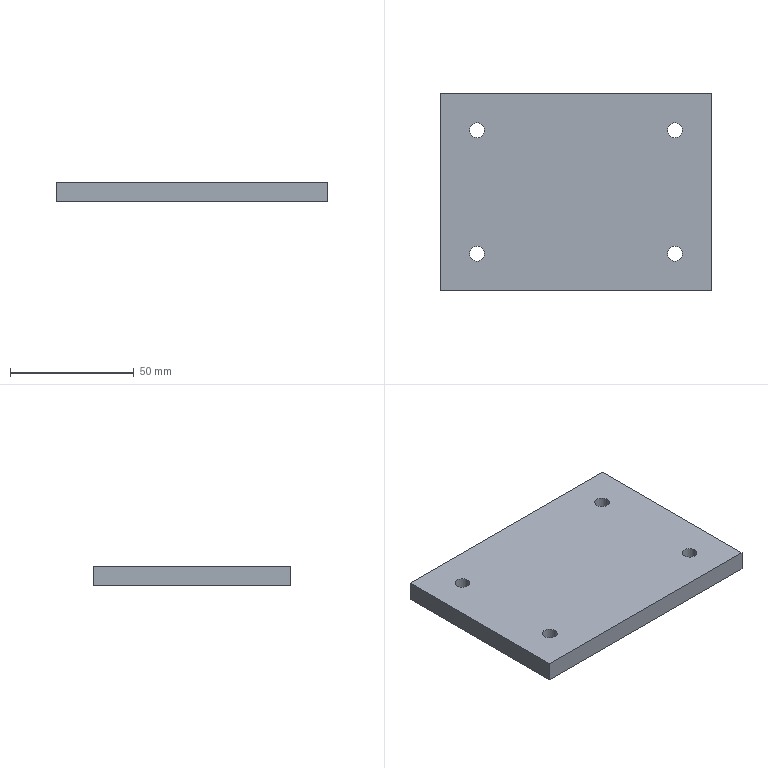Component | NX | 5 | 1 solid | 10 faces | box 110 x 80 x 8 mm | volume 69495 mm3 | plane 6 | cylinder 4 | commonest cylinder face diameters 6 x4
STEP:
#1=CARTESIAN_POINT('',(0.,0.,0.));
#2=DIRECTION('',(0.,0.,1.));
#3=DIRECTION('',(1.,0.,0.));
#4=AXIS2_PLACEMENT_3D('',#1,#2,#3);
#5=CARTESIAN_POINT('',(-55.,40.,0.));
#6=VERTEX_POINT('',#5);
#7=CARTESIAN_POINT('',(-55.,-40.,0.));
#8=VERTEX_POINT('',#7);
#9=CARTESIAN_POINT('',(-55.,40.,0.));
#10=DIRECTION('',(-0.,-1.,0.));
#11=VECTOR('',#10,1.);
#12=LINE('',#9,#11);
#13=CARTESIAN_POINT('',(-55.,40.,-8.));
#14=DIRECTION('',(-1.,0.,0.));
#15=DIRECTION('',(-0.,-1.,0.));
#16=AXIS2_PLACEMENT_3D('',#13,#14,#15);
#17=PLANE('',#16);
#18=CARTESIAN_POINT('',(0.,8.));
#19=DIRECTION('',(1.,0.));
#20=VECTOR('',#19,1.);
#21=LINE('',#18,#20);
#22=(GEOMETRIC_REPRESENTATION_CONTEXT(2)PARAMETRIC_REPRESENTATION_CONTEXT()REPRESENTATION_CONTEXT('',''));
#23=DEFINITIONAL_REPRESENTATION('',(#21),#22);
#24=PCURVE('',#17,#23);
#25=CARTESIAN_POINT('',(0.,0.,0.));
#26=DIRECTION('',(0.,0.,1.));
#27=DIRECTION('',(1.,0.,0.));
#28=AXIS2_PLACEMENT_3D('',#25,#26,#27);
#29=PLANE('',#28);
#30=CARTESIAN_POINT('',(-55.,40.));
#31=DIRECTION('',(-0.,-1.));
#32=VECTOR('',#31,1.);
#33=LINE('',#30,#32);
#34=(GEOMETRIC_REPRESENTATION_CONTEXT(2)PARAMETRIC_REPRESENTATION_CONTEXT()REPRESENTATION_CONTEXT('',''));
#35=DEFINITIONAL_REPRESENTATION('',(#33),#34);
#36=PCURVE('',#29,#35);
#37=SURFACE_CURVE('',#12,(#24,#36),.PCURVE_S1.);
#38=EDGE_CURVE('',#6,#8,#37,.T.);
#39=ORIENTED_EDGE('',*,*,#38,.F.);
#40=CARTESIAN_POINT('',(-55.,40.,-8.));
#41=VERTEX_POINT('',#40);
#42=CARTESIAN_POINT('',(-55.,40.,-8.));
#43=DIRECTION('',(0.,0.,1.));
#44=VECTOR('',#43,1.);
#45=LINE('',#42,#44);
#46=CARTESIAN_POINT('',(0.,0.));
#47=DIRECTION('',(0.,1.));
#48=VECTOR('',#47,1.);
#49=LINE('',#46,#48);
#50=(GEOMETRIC_REPRESENTATION_CONTEXT(2)PARAMETRIC_REPRESENTATION_CONTEXT()REPRESENTATION_CONTEXT('',''));
#51=DEFINITIONAL_REPRESENTATION('',(#49),#50);
#52=PCURVE('',#17,#51);
#53=CARTESIAN_POINT('',(55.,40.,-8.));
#54=DIRECTION('',(0.,1.,0.));
#55=DIRECTION('',(0.,0.,1.));
#56=AXIS2_PLACEMENT_3D('',#53,#54,#55);
#57=PLANE('',#56);
#58=CARTESIAN_POINT('',(0.,-110.));
#59=DIRECTION('',(1.,0.));
#60=VECTOR('',#59,1.);
#61=LINE('',#58,#60);
#62=(GEOMETRIC_REPRESENTATION_CONTEXT(2)PARAMETRIC_REPRESENTATION_CONTEXT()REPRESENTATION_CONTEXT('',''));
#63=DEFINITIONAL_REPRESENTATION('',(#61),#62);
#64=PCURVE('',#57,#63);
#65=SURFACE_CURVE('',#45,(#52,#64),.PCURVE_S1.);
#66=EDGE_CURVE('',#41,#6,#65,.T.);
#67=ORIENTED_EDGE('',*,*,#66,.F.);
#68=CARTESIAN_POINT('',(-55.,-40.,-8.));
#69=VERTEX_POINT('',#68);
#70=CARTESIAN_POINT('',(-55.,40.,-8.));
#71=DIRECTION('',(-0.,-1.,0.));
#72=VECTOR('',#71,1.);
#73=LINE('',#70,#72);
#74=CARTESIAN_POINT('',(0.,0.));
#75=DIRECTION('',(1.,0.));
#76=VECTOR('',#75,1.);
#77=LINE('',#74,#76);
#78=(GEOMETRIC_REPRESENTATION_CONTEXT(2)PARAMETRIC_REPRESENTATION_CONTEXT()REPRESENTATION_CONTEXT('',''));
#79=DEFINITIONAL_REPRESENTATION('',(#77),#78);
#80=PCURVE('',#17,#79);
#81=CARTESIAN_POINT('',(0.,0.,-8.));
#82=DIRECTION('',(0.,0.,1.));
#83=DIRECTION('',(1.,0.,0.));
#84=AXIS2_PLACEMENT_3D('',#81,#82,#83);
#85=PLANE('',#84);
#86=CARTESIAN_POINT('',(-55.,40.));
#87=DIRECTION('',(-0.,-1.));
#88=VECTOR('',#87,1.);
#89=LINE('',#86,#88);
#90=(GEOMETRIC_REPRESENTATION_CONTEXT(2)PARAMETRIC_REPRESENTATION_CONTEXT()REPRESENTATION_CONTEXT('',''));
#91=DEFINITIONAL_REPRESENTATION('',(#89),#90);
#92=PCURVE('',#85,#91);
#93=SURFACE_CURVE('',#73,(#80,#92),.PCURVE_S1.);
#94=EDGE_CURVE('',#41,#69,#93,.T.);
#95=ORIENTED_EDGE('',*,*,#94,.T.);
#96=CARTESIAN_POINT('',(-55.,-40.,-8.));
#97=DIRECTION('',(0.,0.,1.));
#98=VECTOR('',#97,1.);
#99=LINE('',#96,#98);
#100=CARTESIAN_POINT('',(80.,0.));
#101=DIRECTION('',(0.,1.));
#102=VECTOR('',#101,1.);
#103=LINE('',#100,#102);
#104=(GEOMETRIC_REPRESENTATION_CONTEXT(2)PARAMETRIC_REPRESENTATION_CONTEXT()REPRESENTATION_CONTEXT('',''));
#105=DEFINITIONAL_REPRESENTATION('',(#103),#104);
#106=PCURVE('',#17,#105);
#107=CARTESIAN_POINT('',(-55.,-40.,-8.));
#108=DIRECTION('',(0.,-1.,0.));
#109=DIRECTION('',(0.,0.,-1.));
#110=AXIS2_PLACEMENT_3D('',#107,#108,#109);
#111=PLANE('',#110);
#112=CARTESIAN_POINT('',(0.,0.));
#113=DIRECTION('',(-1.,0.));
#114=VECTOR('',#113,1.);
#115=LINE('',#112,#114);
#116=(GEOMETRIC_REPRESENTATION_CONTEXT(2)PARAMETRIC_REPRESENTATION_CONTEXT()REPRESENTATION_CONTEXT('',''));
#117=DEFINITIONAL_REPRESENTATION('',(#115),#116);
#118=PCURVE('',#111,#117);
#119=SURFACE_CURVE('',#99,(#106,#118),.PCURVE_S1.);
#120=EDGE_CURVE('',#69,#8,#119,.T.);
#121=ORIENTED_EDGE('',*,*,#120,.T.);
#122=EDGE_LOOP('',(#39,#67,#95,#121));
#123=FACE_BOUND('',#122,.T.);
#124=ADVANCED_FACE('',(#123),#17,.T.);
#125=CARTESIAN_POINT('',(55.,-40.,0.));
#126=VERTEX_POINT('',#125);
#127=CARTESIAN_POINT('',(-55.,-40.,0.));
#128=DIRECTION('',(1.,0.,0.));
#129=VECTOR('',#128,1.);
#130=LINE('',#127,#129);
#131=CARTESIAN_POINT('',(-8.,0.));
#132=DIRECTION('',(0.,1.));
#133=VECTOR('',#132,1.);
#134=LINE('',#131,#133);
#135=(GEOMETRIC_REPRESENTATION_CONTEXT(2)PARAMETRIC_REPRESENTATION_CONTEXT()REPRESENTATION_CONTEXT('',''));
#136=DEFINITIONAL_REPRESENTATION('',(#134),#135);
#137=PCURVE('',#111,#136);
#138=CARTESIAN_POINT('',(-55.,-40.));
#139=DIRECTION('',(1.,0.));
#140=VECTOR('',#139,1.);
#141=LINE('',#138,#140);
#142=(GEOMETRIC_REPRESENTATION_CONTEXT(2)PARAMETRIC_REPRESENTATION_CONTEXT()REPRESENTATION_CONTEXT('',''));
#143=DEFINITIONAL_REPRESENTATION('',(#141),#142);
#144=PCURVE('',#29,#143);
#145=SURFACE_CURVE('',#130,(#137,#144),.PCURVE_S1.);
#146=EDGE_CURVE('',#8,#126,#145,.T.);
#147=ORIENTED_EDGE('',*,*,#146,.F.);
#148=ORIENTED_EDGE('',*,*,#120,.F.);
#149=CARTESIAN_POINT('',(55.,-40.,-8.));
#150=VERTEX_POINT('',#149);
#151=CARTESIAN_POINT('',(-55.,-40.,-8.));
#152=DIRECTION('',(1.,0.,0.));
#153=VECTOR('',#152,1.);
#154=LINE('',#151,#153);
#155=CARTESIAN_POINT('',(0.,0.));
#156=DIRECTION('',(0.,1.));
#157=VECTOR('',#156,1.);
#158=LINE('',#155,#157);
#159=(GEOMETRIC_REPRESENTATION_CONTEXT(2)PARAMETRIC_REPRESENTATION_CONTEXT()REPRESENTATION_CONTEXT('',''));
#160=DEFINITIONAL_REPRESENTATION('',(#158),#159);
#161=PCURVE('',#111,#160);
#162=CARTESIAN_POINT('',(-55.,-40.));
#163=DIRECTION('',(1.,0.));
#164=VECTOR('',#163,1.);
#165=LINE('',#162,#164);
#166=(GEOMETRIC_REPRESENTATION_CONTEXT(2)PARAMETRIC_REPRESENTATION_CONTEXT()REPRESENTATION_CONTEXT('',''));
#167=DEFINITIONAL_REPRESENTATION('',(#165),#166);
#168=PCURVE('',#85,#167);
#169=SURFACE_CURVE('',#154,(#161,#168),.PCURVE_S1.);
#170=EDGE_CURVE('',#69,#150,#169,.T.);
#171=ORIENTED_EDGE('',*,*,#170,.T.);
#172=CARTESIAN_POINT('',(55.,-40.,-8.));
#173=DIRECTION('',(0.,0.,1.));
#174=VECTOR('',#173,1.);
#175=LINE('',#172,#174);
#176=CARTESIAN_POINT('',(0.,110.));
#177=DIRECTION('',(-1.,0.));
#178=VECTOR('',#177,1.);
#179=LINE('',#176,#178);
#180=(GEOMETRIC_REPRESENTATION_CONTEXT(2)PARAMETRIC_REPRESENTATION_CONTEXT()REPRESENTATION_CONTEXT('',''));
#181=DEFINITIONAL_REPRESENTATION('',(#179),#180);
#182=PCURVE('',#111,#181);
#183=CARTESIAN_POINT('',(55.,-40.,-8.));
#184=DIRECTION('',(1.,0.,0.));
#185=DIRECTION('',(-0.,1.,0.));
#186=AXIS2_PLACEMENT_3D('',#183,#184,#185);
#187=PLANE('',#186);
#188=CARTESIAN_POINT('',(0.,0.));
#189=DIRECTION('',(0.,1.));
#190=VECTOR('',#189,1.);
#191=LINE('',#188,#190);
#192=(GEOMETRIC_REPRESENTATION_CONTEXT(2)PARAMETRIC_REPRESENTATION_CONTEXT()REPRESENTATION_CONTEXT('',''));
#193=DEFINITIONAL_REPRESENTATION('',(#191),#192);
#194=PCURVE('',#187,#193);
#195=SURFACE_CURVE('',#175,(#182,#194),.PCURVE_S1.);
#196=EDGE_CURVE('',#150,#126,#195,.T.);
#197=ORIENTED_EDGE('',*,*,#196,.T.);
#198=EDGE_LOOP('',(#147,#148,#171,#197));
#199=FACE_BOUND('',#198,.T.);
#200=ADVANCED_FACE('',(#199),#111,.T.);
#201=CARTESIAN_POINT('',(55.,40.,0.));
#202=VERTEX_POINT('',#201);
#203=CARTESIAN_POINT('',(55.,-40.,0.));
#204=DIRECTION('',(-0.,1.,0.));
#205=VECTOR('',#204,1.);
#206=LINE('',#203,#205);
#207=CARTESIAN_POINT('',(0.,8.));
#208=DIRECTION('',(1.,0.));
#209=VECTOR('',#208,1.);
#210=LINE('',#207,#209);
#211=(GEOMETRIC_REPRESENTATION_CONTEXT(2)PARAMETRIC_REPRESENTATION_CONTEXT()REPRESENTATION_CONTEXT('',''));
#212=DEFINITIONAL_REPRESENTATION('',(#210),#211);
#213=PCURVE('',#187,#212);
#214=CARTESIAN_POINT('',(55.,-40.));
#215=DIRECTION('',(-0.,1.));
#216=VECTOR('',#215,1.);
#217=LINE('',#214,#216);
#218=(GEOMETRIC_REPRESENTATION_CONTEXT(2)PARAMETRIC_REPRESENTATION_CONTEXT()REPRESENTATION_CONTEXT('',''));
#219=DEFINITIONAL_REPRESENTATION('',(#217),#218);
#220=PCURVE('',#29,#219);
#221=SURFACE_CURVE('',#206,(#213,#220),.PCURVE_S1.);
#222=EDGE_CURVE('',#126,#202,#221,.T.);
#223=ORIENTED_EDGE('',*,*,#222,.F.);
#224=ORIENTED_EDGE('',*,*,#196,.F.);
#225=CARTESIAN_POINT('',(55.,40.,-8.));
#226=VERTEX_POINT('',#225);
#227=CARTESIAN_POINT('',(55.,-40.,-8.));
#228=DIRECTION('',(-0.,1.,0.));
#229=VECTOR('',#228,1.);
#230=LINE('',#227,#229);
#231=CARTESIAN_POINT('',(0.,0.));
#232=DIRECTION('',(1.,0.));
#233=VECTOR('',#232,1.);
#234=LINE('',#231,#233);
#235=(GEOMETRIC_REPRESENTATION_CONTEXT(2)PARAMETRIC_REPRESENTATION_CONTEXT()REPRESENTATION_CONTEXT('',''));
#236=DEFINITIONAL_REPRESENTATION('',(#234),#235);
#237=PCURVE('',#187,#236);
#238=CARTESIAN_POINT('',(55.,-40.));
#239=DIRECTION('',(-0.,1.));
#240=VECTOR('',#239,1.);
#241=LINE('',#238,#240);
#242=(GEOMETRIC_REPRESENTATION_CONTEXT(2)PARAMETRIC_REPRESENTATION_CONTEXT()REPRESENTATION_CONTEXT('',''));
#243=DEFINITIONAL_REPRESENTATION('',(#241),#242);
#244=PCURVE('',#85,#243);
#245=SURFACE_CURVE('',#230,(#237,#244),.PCURVE_S1.);
#246=EDGE_CURVE('',#150,#226,#245,.T.);
#247=ORIENTED_EDGE('',*,*,#246,.T.);
#248=CARTESIAN_POINT('',(55.,40.,-8.));
#249=DIRECTION('',(0.,0.,1.));
#250=VECTOR('',#249,1.);
#251=LINE('',#248,#250);
#252=CARTESIAN_POINT('',(80.,0.));
#253=DIRECTION('',(0.,1.));
#254=VECTOR('',#253,1.);
#255=LINE('',#252,#254);
#256=(GEOMETRIC_REPRESENTATION_CONTEXT(2)PARAMETRIC_REPRESENTATION_CONTEXT()REPRESENTATION_CONTEXT('',''));
#257=DEFINITIONAL_REPRESENTATION('',(#255),#256);
#258=PCURVE('',#187,#257);
#259=CARTESIAN_POINT('',(0.,0.));
#260=DIRECTION('',(1.,0.));
#261=VECTOR('',#260,1.);
#262=LINE('',#259,#261);
#263=(GEOMETRIC_REPRESENTATION_CONTEXT(2)PARAMETRIC_REPRESENTATION_CONTEXT()REPRESENTATION_CONTEXT('',''));
#264=DEFINITIONAL_REPRESENTATION('',(#262),#263);
#265=PCURVE('',#57,#264);
#266=SURFACE_CURVE('',#251,(#258,#265),.PCURVE_S1.);
#267=EDGE_CURVE('',#226,#202,#266,.T.);
#268=ORIENTED_EDGE('',*,*,#267,.T.);
#269=EDGE_LOOP('',(#223,#224,#247,#268));
#270=FACE_BOUND('',#269,.T.);
#271=ADVANCED_FACE('',(#270),#187,.T.);
#272=CARTESIAN_POINT('',(55.,40.,0.));
#273=DIRECTION('',(-1.,0.,0.));
#274=VECTOR('',#273,1.);
#275=LINE('',#272,#274);
#276=CARTESIAN_POINT('',(8.,0.));
#277=DIRECTION('',(0.,-1.));
#278=VECTOR('',#277,1.);
#279=LINE('',#276,#278);
#280=(GEOMETRIC_REPRESENTATION_CONTEXT(2)PARAMETRIC_REPRESENTATION_CONTEXT()REPRESENTATION_CONTEXT('',''));
#281=DEFINITIONAL_REPRESENTATION('',(#279),#280);
#282=PCURVE('',#57,#281);
#283=CARTESIAN_POINT('',(55.,40.));
#284=DIRECTION('',(-1.,0.));
#285=VECTOR('',#284,1.);
#286=LINE('',#283,#285);
#287=(GEOMETRIC_REPRESENTATION_CONTEXT(2)PARAMETRIC_REPRESENTATION_CONTEXT()REPRESENTATION_CONTEXT('',''));
#288=DEFINITIONAL_REPRESENTATION('',(#286),#287);
#289=PCURVE('',#29,#288);
#290=SURFACE_CURVE('',#275,(#282,#289),.PCURVE_S1.);
#291=EDGE_CURVE('',#202,#6,#290,.T.);
#292=ORIENTED_EDGE('',*,*,#291,.F.);
#293=ORIENTED_EDGE('',*,*,#267,.F.);
#294=CARTESIAN_POINT('',(55.,40.,-8.));
#295=DIRECTION('',(-1.,0.,0.));
#296=VECTOR('',#295,1.);
#297=LINE('',#294,#296);
#298=CARTESIAN_POINT('',(0.,0.));
#299=DIRECTION('',(0.,-1.));
#300=VECTOR('',#299,1.);
#301=LINE('',#298,#300);
#302=(GEOMETRIC_REPRESENTATION_CONTEXT(2)PARAMETRIC_REPRESENTATION_CONTEXT()REPRESENTATION_CONTEXT('',''));
#303=DEFINITIONAL_REPRESENTATION('',(#301),#302);
#304=PCURVE('',#57,#303);
#305=CARTESIAN_POINT('',(55.,40.));
#306=DIRECTION('',(-1.,0.));
#307=VECTOR('',#306,1.);
#308=LINE('',#305,#307);
#309=(GEOMETRIC_REPRESENTATION_CONTEXT(2)PARAMETRIC_REPRESENTATION_CONTEXT()REPRESENTATION_CONTEXT('',''));
#310=DEFINITIONAL_REPRESENTATION('',(#308),#309);
#311=PCURVE('',#85,#310);
#312=SURFACE_CURVE('',#297,(#304,#311),.PCURVE_S1.);
#313=EDGE_CURVE('',#226,#41,#312,.T.);
#314=ORIENTED_EDGE('',*,*,#313,.T.);
#315=ORIENTED_EDGE('',*,*,#66,.T.);
#316=EDGE_LOOP('',(#292,#293,#314,#315));
#317=FACE_BOUND('',#316,.T.);
#318=ADVANCED_FACE('',(#317),#57,.T.);
#319=CARTESIAN_POINT('',(43.,25.,-8.));
#320=VERTEX_POINT('',#319);
#321=CARTESIAN_POINT('',(37.,25.,-8.));
#322=VERTEX_POINT('',#321);
#323=CARTESIAN_POINT('',(40.,25.,-8.));
#324=DIRECTION('',(0.,0.,1.));
#325=DIRECTION('',(1.,0.,0.));
#326=AXIS2_PLACEMENT_3D('',#323,#324,#325);
#327=CIRCLE('',#326,3.);
#328=CARTESIAN_POINT('',(40.,25.));
#329=DIRECTION('',(1.,0.));
#330=AXIS2_PLACEMENT_2D('',#328,#329);
#331=CIRCLE('',#330,3.);
#332=(GEOMETRIC_REPRESENTATION_CONTEXT(2)PARAMETRIC_REPRESENTATION_CONTEXT()REPRESENTATION_CONTEXT('',''));
#333=DEFINITIONAL_REPRESENTATION('',(#331),#332);
#334=PCURVE('',#85,#333);
#335=CARTESIAN_POINT('',(40.,25.,0.));
#336=DIRECTION('',(0.,0.,-1.));
#337=DIRECTION('',(-1.,0.,0.));
#338=AXIS2_PLACEMENT_3D('',#335,#336,#337);
#339=CYLINDRICAL_SURFACE('',#338,3.);
#340=CARTESIAN_POINT('',(3.142,8.));
#341=DIRECTION('',(-1.,0.));
#342=VECTOR('',#341,1.);
#343=LINE('',#340,#342);
#344=(GEOMETRIC_REPRESENTATION_CONTEXT(2)PARAMETRIC_REPRESENTATION_CONTEXT()REPRESENTATION_CONTEXT('',''));
#345=DEFINITIONAL_REPRESENTATION('',(#343),#344);
#346=PCURVE('',#339,#345);
#347=SURFACE_CURVE('',#327,(#334,#346),.PCURVE_S1.);
#348=EDGE_CURVE('',#320,#322,#347,.T.);
#349=ORIENTED_EDGE('',*,*,#348,.T.);
#350=CARTESIAN_POINT('',(40.,25.,-8.));
#351=DIRECTION('',(0.,0.,1.));
#352=DIRECTION('',(1.,0.,0.));
#353=AXIS2_PLACEMENT_3D('',#350,#351,#352);
#354=CIRCLE('',#353,3.);
#355=CARTESIAN_POINT('',(40.,25.));
#356=DIRECTION('',(1.,0.));
#357=AXIS2_PLACEMENT_2D('',#355,#356);
#358=CIRCLE('',#357,3.);
#359=(GEOMETRIC_REPRESENTATION_CONTEXT(2)PARAMETRIC_REPRESENTATION_CONTEXT()REPRESENTATION_CONTEXT('',''));
#360=DEFINITIONAL_REPRESENTATION('',(#358),#359);
#361=PCURVE('',#85,#360);
#362=CARTESIAN_POINT('',(9.425,8.));
#363=DIRECTION('',(-1.,0.));
#364=VECTOR('',#363,1.);
#365=LINE('',#362,#364);
#366=(GEOMETRIC_REPRESENTATION_CONTEXT(2)PARAMETRIC_REPRESENTATION_CONTEXT()REPRESENTATION_CONTEXT('',''));
#367=DEFINITIONAL_REPRESENTATION('',(#365),#366);
#368=PCURVE('',#339,#367);
#369=SURFACE_CURVE('',#354,(#361,#368),.PCURVE_S1.);
#370=EDGE_CURVE('',#322,#320,#369,.T.);
#371=ORIENTED_EDGE('',*,*,#370,.T.);
#372=EDGE_LOOP('',(#349,#371));
#373=FACE_BOUND('',#372,.T.);
#374=CARTESIAN_POINT('',(43.,-25.,-8.));
#375=VERTEX_POINT('',#374);
#376=CARTESIAN_POINT('',(37.,-25.,-8.));
#377=VERTEX_POINT('',#376);
#378=CARTESIAN_POINT('',(40.,-25.,-8.));
#379=DIRECTION('',(0.,0.,1.));
#380=DIRECTION('',(1.,0.,0.));
#381=AXIS2_PLACEMENT_3D('',#378,#379,#380);
#382=CIRCLE('',#381,3.);
#383=CARTESIAN_POINT('',(40.,-25.));
#384=DIRECTION('',(1.,0.));
#385=AXIS2_PLACEMENT_2D('',#383,#384);
#386=CIRCLE('',#385,3.);
#387=(GEOMETRIC_REPRESENTATION_CONTEXT(2)PARAMETRIC_REPRESENTATION_CONTEXT()REPRESENTATION_CONTEXT('',''));
#388=DEFINITIONAL_REPRESENTATION('',(#386),#387);
#389=PCURVE('',#85,#388);
#390=CARTESIAN_POINT('',(40.,-25.,0.));
#391=DIRECTION('',(0.,0.,-1.));
#392=DIRECTION('',(-1.,0.,0.));
#393=AXIS2_PLACEMENT_3D('',#390,#391,#392);
#394=CYLINDRICAL_SURFACE('',#393,3.);
#395=CARTESIAN_POINT('',(3.142,8.));
#396=DIRECTION('',(-1.,0.));
#397=VECTOR('',#396,1.);
#398=LINE('',#395,#397);
#399=(GEOMETRIC_REPRESENTATION_CONTEXT(2)PARAMETRIC_REPRESENTATION_CONTEXT()REPRESENTATION_CONTEXT('',''));
#400=DEFINITIONAL_REPRESENTATION('',(#398),#399);
#401=PCURVE('',#394,#400);
#402=SURFACE_CURVE('',#382,(#389,#401),.PCURVE_S1.);
#403=EDGE_CURVE('',#375,#377,#402,.T.);
#404=ORIENTED_EDGE('',*,*,#403,.T.);
#405=CARTESIAN_POINT('',(40.,-25.,-8.));
#406=DIRECTION('',(0.,0.,1.));
#407=DIRECTION('',(1.,0.,0.));
#408=AXIS2_PLACEMENT_3D('',#405,#406,#407);
#409=CIRCLE('',#408,3.);
#410=CARTESIAN_POINT('',(40.,-25.));
#411=DIRECTION('',(1.,0.));
#412=AXIS2_PLACEMENT_2D('',#410,#411);
#413=CIRCLE('',#412,3.);
#414=(GEOMETRIC_REPRESENTATION_CONTEXT(2)PARAMETRIC_REPRESENTATION_CONTEXT()REPRESENTATION_CONTEXT('',''));
#415=DEFINITIONAL_REPRESENTATION('',(#413),#414);
#416=PCURVE('',#85,#415);
#417=CARTESIAN_POINT('',(9.425,8.));
#418=DIRECTION('',(-1.,0.));
#419=VECTOR('',#418,1.);
#420=LINE('',#417,#419);
#421=(GEOMETRIC_REPRESENTATION_CONTEXT(2)PARAMETRIC_REPRESENTATION_CONTEXT()REPRESENTATION_CONTEXT('',''));
#422=DEFINITIONAL_REPRESENTATION('',(#420),#421);
#423=PCURVE('',#394,#422);
#424=SURFACE_CURVE('',#409,(#416,#423),.PCURVE_S1.);
#425=EDGE_CURVE('',#377,#375,#424,.T.);
#426=ORIENTED_EDGE('',*,*,#425,.T.);
#427=EDGE_LOOP('',(#404,#426));
#428=FACE_BOUND('',#427,.T.);
#429=CARTESIAN_POINT('',(-37.,25.,-8.));
#430=VERTEX_POINT('',#429);
#431=CARTESIAN_POINT('',(-43.,25.,-8.));
#432=VERTEX_POINT('',#431);
#433=CARTESIAN_POINT('',(-40.,25.,-8.));
#434=DIRECTION('',(0.,0.,1.));
#435=DIRECTION('',(1.,0.,0.));
#436=AXIS2_PLACEMENT_3D('',#433,#434,#435);
#437=CIRCLE('',#436,3.);
#438=CARTESIAN_POINT('',(-40.,25.));
#439=DIRECTION('',(1.,0.));
#440=AXIS2_PLACEMENT_2D('',#438,#439);
#441=CIRCLE('',#440,3.);
#442=(GEOMETRIC_REPRESENTATION_CONTEXT(2)PARAMETRIC_REPRESENTATION_CONTEXT()REPRESENTATION_CONTEXT('',''));
#443=DEFINITIONAL_REPRESENTATION('',(#441),#442);
#444=PCURVE('',#85,#443);
#445=CARTESIAN_POINT('',(-40.,25.,0.));
#446=DIRECTION('',(0.,0.,-1.));
#447=DIRECTION('',(-1.,0.,0.));
#448=AXIS2_PLACEMENT_3D('',#445,#446,#447);
#449=CYLINDRICAL_SURFACE('',#448,3.);
#450=CARTESIAN_POINT('',(3.142,8.));
#451=DIRECTION('',(-1.,0.));
#452=VECTOR('',#451,1.);
#453=LINE('',#450,#452);
#454=(GEOMETRIC_REPRESENTATION_CONTEXT(2)PARAMETRIC_REPRESENTATION_CONTEXT()REPRESENTATION_CONTEXT('',''));
#455=DEFINITIONAL_REPRESENTATION('',(#453),#454);
#456=PCURVE('',#449,#455);
#457=SURFACE_CURVE('',#437,(#444,#456),.PCURVE_S1.);
#458=EDGE_CURVE('',#430,#432,#457,.T.);
#459=ORIENTED_EDGE('',*,*,#458,.T.);
#460=CARTESIAN_POINT('',(-40.,25.,-8.));
#461=DIRECTION('',(0.,0.,1.));
#462=DIRECTION('',(1.,0.,0.));
#463=AXIS2_PLACEMENT_3D('',#460,#461,#462);
#464=CIRCLE('',#463,3.);
#465=CARTESIAN_POINT('',(-40.,25.));
#466=DIRECTION('',(1.,0.));
#467=AXIS2_PLACEMENT_2D('',#465,#466);
#468=CIRCLE('',#467,3.);
#469=(GEOMETRIC_REPRESENTATION_CONTEXT(2)PARAMETRIC_REPRESENTATION_CONTEXT()REPRESENTATION_CONTEXT('',''));
#470=DEFINITIONAL_REPRESENTATION('',(#468),#469);
#471=PCURVE('',#85,#470);
#472=CARTESIAN_POINT('',(9.425,8.));
#473=DIRECTION('',(-1.,0.));
#474=VECTOR('',#473,1.);
#475=LINE('',#472,#474);
#476=(GEOMETRIC_REPRESENTATION_CONTEXT(2)PARAMETRIC_REPRESENTATION_CONTEXT()REPRESENTATION_CONTEXT('',''));
#477=DEFINITIONAL_REPRESENTATION('',(#475),#476);
#478=PCURVE('',#449,#477);
#479=SURFACE_CURVE('',#464,(#471,#478),.PCURVE_S1.);
#480=EDGE_CURVE('',#432,#430,#479,.T.);
#481=ORIENTED_EDGE('',*,*,#480,.T.);
#482=EDGE_LOOP('',(#459,#481));
#483=FACE_BOUND('',#482,.T.);
#484=CARTESIAN_POINT('',(-37.,-25.,-8.));
#485=VERTEX_POINT('',#484);
#486=CARTESIAN_POINT('',(-43.,-25.,-8.));
#487=VERTEX_POINT('',#486);
#488=CARTESIAN_POINT('',(-40.,-25.,-8.));
#489=DIRECTION('',(0.,0.,1.));
#490=DIRECTION('',(1.,0.,0.));
#491=AXIS2_PLACEMENT_3D('',#488,#489,#490);
#492=CIRCLE('',#491,3.);
#493=CARTESIAN_POINT('',(-40.,-25.));
#494=DIRECTION('',(1.,0.));
#495=AXIS2_PLACEMENT_2D('',#493,#494);
#496=CIRCLE('',#495,3.);
#497=(GEOMETRIC_REPRESENTATION_CONTEXT(2)PARAMETRIC_REPRESENTATION_CONTEXT()REPRESENTATION_CONTEXT('',''));
#498=DEFINITIONAL_REPRESENTATION('',(#496),#497);
#499=PCURVE('',#85,#498);
#500=CARTESIAN_POINT('',(-40.,-25.,0.));
#501=DIRECTION('',(0.,0.,-1.));
#502=DIRECTION('',(-1.,0.,0.));
#503=AXIS2_PLACEMENT_3D('',#500,#501,#502);
#504=CYLINDRICAL_SURFACE('',#503,3.);
#505=CARTESIAN_POINT('',(3.142,8.));
#506=DIRECTION('',(-1.,0.));
#507=VECTOR('',#506,1.);
#508=LINE('',#505,#507);
#509=(GEOMETRIC_REPRESENTATION_CONTEXT(2)PARAMETRIC_REPRESENTATION_CONTEXT()REPRESENTATION_CONTEXT('',''));
#510=DEFINITIONAL_REPRESENTATION('',(#508),#509);
#511=PCURVE('',#504,#510);
#512=SURFACE_CURVE('',#492,(#499,#511),.PCURVE_S1.);
#513=EDGE_CURVE('',#485,#487,#512,.T.);
#514=ORIENTED_EDGE('',*,*,#513,.T.);
#515=CARTESIAN_POINT('',(-40.,-25.,-8.));
#516=DIRECTION('',(0.,0.,1.));
#517=DIRECTION('',(1.,0.,0.));
#518=AXIS2_PLACEMENT_3D('',#515,#516,#517);
#519=CIRCLE('',#518,3.);
#520=CARTESIAN_POINT('',(-40.,-25.));
#521=DIRECTION('',(1.,0.));
#522=AXIS2_PLACEMENT_2D('',#520,#521);
#523=CIRCLE('',#522,3.);
#524=(GEOMETRIC_REPRESENTATION_CONTEXT(2)PARAMETRIC_REPRESENTATION_CONTEXT()REPRESENTATION_CONTEXT('',''));
#525=DEFINITIONAL_REPRESENTATION('',(#523),#524);
#526=PCURVE('',#85,#525);
#527=CARTESIAN_POINT('',(9.425,8.));
#528=DIRECTION('',(-1.,0.));
#529=VECTOR('',#528,1.);
#530=LINE('',#527,#529);
#531=(GEOMETRIC_REPRESENTATION_CONTEXT(2)PARAMETRIC_REPRESENTATION_CONTEXT()REPRESENTATION_CONTEXT('',''));
#532=DEFINITIONAL_REPRESENTATION('',(#530),#531);
#533=PCURVE('',#504,#532);
#534=SURFACE_CURVE('',#519,(#526,#533),.PCURVE_S1.);
#535=EDGE_CURVE('',#487,#485,#534,.T.);
#536=ORIENTED_EDGE('',*,*,#535,.T.);
#537=EDGE_LOOP('',(#514,#536));
#538=FACE_BOUND('',#537,.T.);
#539=ORIENTED_EDGE('',*,*,#94,.F.);
#540=ORIENTED_EDGE('',*,*,#313,.F.);
#541=ORIENTED_EDGE('',*,*,#246,.F.);
#542=ORIENTED_EDGE('',*,*,#170,.F.);
#543=EDGE_LOOP('',(#539,#540,#541,#542));
#544=FACE_BOUND('',#543,.T.);
#545=ADVANCED_FACE('',(#373,#428,#483,#538,#544),#85,.F.);
#546=CARTESIAN_POINT('',(37.,25.,0.));
#547=VERTEX_POINT('',#546);
#548=CARTESIAN_POINT('',(40.,25.,0.));
#549=DIRECTION('',(0.,0.,-1.));
#550=DIRECTION('',(-1.,0.,0.));
#551=AXIS2_PLACEMENT_3D('',#548,#549,#550);
#552=CIRCLE('',#551,3.);
#553=CARTESIAN_POINT('',(37.,25.));
#554=CARTESIAN_POINT('',(37.,30.196));
#555=CARTESIAN_POINT('',(41.5,27.598));
#556=CARTESIAN_POINT('',(46.,25.));
#557=CARTESIAN_POINT('',(41.5,22.402));
#558=CARTESIAN_POINT('',(37.,19.804));
#559=CARTESIAN_POINT('',(37.,25.));
#560=(BOUNDED_CURVE()B_SPLINE_CURVE(2,(#553,#554,#555,#556,#557,#558,#559),.UNSPECIFIED.,.T.,.F.)B_SPLINE_CURVE_WITH_KNOTS((1,2,2,2,2,1),(-2.094,0.,2.094,4.189,6.283,8.378),.UNSPECIFIED.)CURVE()GEOMETRIC_REPRESENTATION_ITEM()RATIONAL_B_SPLINE_CURVE((1.,0.5,1.,0.5,1.,0.5,1.))REPRESENTATION_ITEM(''));
#561=(GEOMETRIC_REPRESENTATION_CONTEXT(2)PARAMETRIC_REPRESENTATION_CONTEXT()REPRESENTATION_CONTEXT('',''));
#562=DEFINITIONAL_REPRESENTATION('',(#560),#561);
#563=PCURVE('',#29,#562);
#564=CARTESIAN_POINT('',(0.,0.));
#565=DIRECTION('',(1.,0.));
#566=VECTOR('',#565,1.);
#567=LINE('',#564,#566);
#568=(GEOMETRIC_REPRESENTATION_CONTEXT(2)PARAMETRIC_REPRESENTATION_CONTEXT()REPRESENTATION_CONTEXT('',''));
#569=DEFINITIONAL_REPRESENTATION('',(#567),#568);
#570=PCURVE('',#339,#569);
#571=SURFACE_CURVE('',#552,(#563,#570),.PCURVE_S1.);
#572=EDGE_CURVE('',#547,#547,#571,.T.);
#573=ORIENTED_EDGE('',*,*,#572,.T.);
#574=EDGE_LOOP('',(#573));
#575=FACE_BOUND('',#574,.T.);
#576=CARTESIAN_POINT('',(37.,-25.,0.));
#577=VERTEX_POINT('',#576);
#578=CARTESIAN_POINT('',(40.,-25.,0.));
#579=DIRECTION('',(0.,0.,-1.));
#580=DIRECTION('',(-1.,0.,0.));
#581=AXIS2_PLACEMENT_3D('',#578,#579,#580);
#582=CIRCLE('',#581,3.);
#583=CARTESIAN_POINT('',(37.,-25.));
#584=CARTESIAN_POINT('',(37.,-19.804));
#585=CARTESIAN_POINT('',(41.5,-22.402));
#586=CARTESIAN_POINT('',(46.,-25.));
#587=CARTESIAN_POINT('',(41.5,-27.598));
#588=CARTESIAN_POINT('',(37.,-30.196));
#589=CARTESIAN_POINT('',(37.,-25.));
#590=(BOUNDED_CURVE()B_SPLINE_CURVE(2,(#583,#584,#585,#586,#587,#588,#589),.UNSPECIFIED.,.T.,.F.)B_SPLINE_CURVE_WITH_KNOTS((1,2,2,2,2,1),(-2.094,0.,2.094,4.189,6.283,8.378),.UNSPECIFIED.)CURVE()GEOMETRIC_REPRESENTATION_ITEM()RATIONAL_B_SPLINE_CURVE((1.,0.5,1.,0.5,1.,0.5,1.))REPRESENTATION_ITEM(''));
#591=(GEOMETRIC_REPRESENTATION_CONTEXT(2)PARAMETRIC_REPRESENTATION_CONTEXT()REPRESENTATION_CONTEXT('',''));
#592=DEFINITIONAL_REPRESENTATION('',(#590),#591);
#593=PCURVE('',#29,#592);
#594=CARTESIAN_POINT('',(0.,0.));
#595=DIRECTION('',(1.,0.));
#596=VECTOR('',#595,1.);
#597=LINE('',#594,#596);
#598=(GEOMETRIC_REPRESENTATION_CONTEXT(2)PARAMETRIC_REPRESENTATION_CONTEXT()REPRESENTATION_CONTEXT('',''));
#599=DEFINITIONAL_REPRESENTATION('',(#597),#598);
#600=PCURVE('',#394,#599);
#601=SURFACE_CURVE('',#582,(#593,#600),.PCURVE_S1.);
#602=EDGE_CURVE('',#577,#577,#601,.T.);
#603=ORIENTED_EDGE('',*,*,#602,.T.);
#604=EDGE_LOOP('',(#603));
#605=FACE_BOUND('',#604,.T.);
#606=CARTESIAN_POINT('',(-43.,25.,0.));
#607=VERTEX_POINT('',#606);
#608=CARTESIAN_POINT('',(-40.,25.,0.));
#609=DIRECTION('',(0.,0.,-1.));
#610=DIRECTION('',(-1.,0.,0.));
#611=AXIS2_PLACEMENT_3D('',#608,#609,#610);
#612=CIRCLE('',#611,3.);
#613=CARTESIAN_POINT('',(-43.,25.));
#614=CARTESIAN_POINT('',(-43.,30.196));
#615=CARTESIAN_POINT('',(-38.5,27.598));
#616=CARTESIAN_POINT('',(-34.,25.));
#617=CARTESIAN_POINT('',(-38.5,22.402));
#618=CARTESIAN_POINT('',(-43.,19.804));
#619=CARTESIAN_POINT('',(-43.,25.));
#620=(BOUNDED_CURVE()B_SPLINE_CURVE(2,(#613,#614,#615,#616,#617,#618,#619),.UNSPECIFIED.,.T.,.F.)B_SPLINE_CURVE_WITH_KNOTS((1,2,2,2,2,1),(-2.094,0.,2.094,4.189,6.283,8.378),.UNSPECIFIED.)CURVE()GEOMETRIC_REPRESENTATION_ITEM()RATIONAL_B_SPLINE_CURVE((1.,0.5,1.,0.5,1.,0.5,1.))REPRESENTATION_ITEM(''));
#621=(GEOMETRIC_REPRESENTATION_CONTEXT(2)PARAMETRIC_REPRESENTATION_CONTEXT()REPRESENTATION_CONTEXT('',''));
#622=DEFINITIONAL_REPRESENTATION('',(#620),#621);
#623=PCURVE('',#29,#622);
#624=CARTESIAN_POINT('',(0.,0.));
#625=DIRECTION('',(1.,0.));
#626=VECTOR('',#625,1.);
#627=LINE('',#624,#626);
#628=(GEOMETRIC_REPRESENTATION_CONTEXT(2)PARAMETRIC_REPRESENTATION_CONTEXT()REPRESENTATION_CONTEXT('',''));
#629=DEFINITIONAL_REPRESENTATION('',(#627),#628);
#630=PCURVE('',#449,#629);
#631=SURFACE_CURVE('',#612,(#623,#630),.PCURVE_S1.);
#632=EDGE_CURVE('',#607,#607,#631,.T.);
#633=ORIENTED_EDGE('',*,*,#632,.T.);
#634=EDGE_LOOP('',(#633));
#635=FACE_BOUND('',#634,.T.);
#636=CARTESIAN_POINT('',(-43.,-25.,0.));
#637=VERTEX_POINT('',#636);
#638=CARTESIAN_POINT('',(-40.,-25.,0.));
#639=DIRECTION('',(0.,0.,-1.));
#640=DIRECTION('',(-1.,0.,0.));
#641=AXIS2_PLACEMENT_3D('',#638,#639,#640);
#642=CIRCLE('',#641,3.);
#643=CARTESIAN_POINT('',(-43.,-25.));
#644=CARTESIAN_POINT('',(-43.,-19.804));
#645=CARTESIAN_POINT('',(-38.5,-22.402));
#646=CARTESIAN_POINT('',(-34.,-25.));
#647=CARTESIAN_POINT('',(-38.5,-27.598));
#648=CARTESIAN_POINT('',(-43.,-30.196));
#649=CARTESIAN_POINT('',(-43.,-25.));
#650=(BOUNDED_CURVE()B_SPLINE_CURVE(2,(#643,#644,#645,#646,#647,#648,#649),.UNSPECIFIED.,.T.,.F.)B_SPLINE_CURVE_WITH_KNOTS((1,2,2,2,2,1),(-2.094,0.,2.094,4.189,6.283,8.378),.UNSPECIFIED.)CURVE()GEOMETRIC_REPRESENTATION_ITEM()RATIONAL_B_SPLINE_CURVE((1.,0.5,1.,0.5,1.,0.5,1.))REPRESENTATION_ITEM(''));
#651=(GEOMETRIC_REPRESENTATION_CONTEXT(2)PARAMETRIC_REPRESENTATION_CONTEXT()REPRESENTATION_CONTEXT('',''));
#652=DEFINITIONAL_REPRESENTATION('',(#650),#651);
#653=PCURVE('',#29,#652);
#654=CARTESIAN_POINT('',(0.,0.));
#655=DIRECTION('',(1.,0.));
#656=VECTOR('',#655,1.);
#657=LINE('',#654,#656);
#658=(GEOMETRIC_REPRESENTATION_CONTEXT(2)PARAMETRIC_REPRESENTATION_CONTEXT()REPRESENTATION_CONTEXT('',''));
#659=DEFINITIONAL_REPRESENTATION('',(#657),#658);
#660=PCURVE('',#504,#659);
#661=SURFACE_CURVE('',#642,(#653,#660),.PCURVE_S1.);
#662=EDGE_CURVE('',#637,#637,#661,.T.);
#663=ORIENTED_EDGE('',*,*,#662,.T.);
#664=EDGE_LOOP('',(#663));
#665=FACE_BOUND('',#664,.T.);
#666=ORIENTED_EDGE('',*,*,#38,.T.);
#667=ORIENTED_EDGE('',*,*,#146,.T.);
#668=ORIENTED_EDGE('',*,*,#222,.T.);
#669=ORIENTED_EDGE('',*,*,#291,.T.);
#670=EDGE_LOOP('',(#666,#667,#668,#669));
#671=FACE_BOUND('',#670,.T.);
#672=ADVANCED_FACE('',(#575,#605,#635,#665,#671),#29,.T.);
#673=ORIENTED_EDGE('',*,*,#662,.T.);
#674=CARTESIAN_POINT('',(-43.,-25.,0.));
#675=CARTESIAN_POINT('',(-43.,-25.,-8.));
#676=B_SPLINE_CURVE_WITH_KNOTS('',1,(#674,#675),.UNSPECIFIED.,.F.,.F.,(2,2),(0.,8.),.PIECEWISE_BEZIER_KNOTS.);
#677=CARTESIAN_POINT('',(6.283,0.));
#678=DIRECTION('',(0.,1.));
#679=VECTOR('',#678,1.);
#680=LINE('',#677,#679);
#681=(GEOMETRIC_REPRESENTATION_CONTEXT(2)PARAMETRIC_REPRESENTATION_CONTEXT()REPRESENTATION_CONTEXT('',''));
#682=DEFINITIONAL_REPRESENTATION('',(#680),#681);
#683=PCURVE('',#504,#682);
#684=CARTESIAN_POINT('',(0.,0.));
#685=DIRECTION('',(0.,1.));
#686=VECTOR('',#685,1.);
#687=LINE('',#684,#686);
#688=(GEOMETRIC_REPRESENTATION_CONTEXT(2)PARAMETRIC_REPRESENTATION_CONTEXT()REPRESENTATION_CONTEXT('',''));
#689=DEFINITIONAL_REPRESENTATION('',(#687),#688);
#690=PCURVE('',#504,#689);
#691=SEAM_CURVE('',#676,(#683,#690),.PCURVE_S1.);
#692=EDGE_CURVE('',#637,#487,#691,.T.);
#693=ORIENTED_EDGE('',*,*,#692,.T.);
#694=ORIENTED_EDGE('',*,*,#535,.T.);
#695=ORIENTED_EDGE('',*,*,#513,.T.);
#696=ORIENTED_EDGE('',*,*,#692,.F.);
#697=EDGE_LOOP('',(#673,#693,#694,#695,#696));
#698=FACE_BOUND('',#697,.F.);
#699=ADVANCED_FACE('',(#698),#504,.F.);
#700=ORIENTED_EDGE('',*,*,#632,.T.);
#701=CARTESIAN_POINT('',(-43.,25.,0.));
#702=CARTESIAN_POINT('',(-43.,25.,-8.));
#703=B_SPLINE_CURVE_WITH_KNOTS('',1,(#701,#702),.UNSPECIFIED.,.F.,.F.,(2,2),(0.,8.),.PIECEWISE_BEZIER_KNOTS.);
#704=CARTESIAN_POINT('',(6.283,0.));
#705=DIRECTION('',(0.,1.));
#706=VECTOR('',#705,1.);
#707=LINE('',#704,#706);
#708=(GEOMETRIC_REPRESENTATION_CONTEXT(2)PARAMETRIC_REPRESENTATION_CONTEXT()REPRESENTATION_CONTEXT('',''));
#709=DEFINITIONAL_REPRESENTATION('',(#707),#708);
#710=PCURVE('',#449,#709);
#711=CARTESIAN_POINT('',(0.,0.));
#712=DIRECTION('',(0.,1.));
#713=VECTOR('',#712,1.);
#714=LINE('',#711,#713);
#715=(GEOMETRIC_REPRESENTATION_CONTEXT(2)PARAMETRIC_REPRESENTATION_CONTEXT()REPRESENTATION_CONTEXT('',''));
#716=DEFINITIONAL_REPRESENTATION('',(#714),#715);
#717=PCURVE('',#449,#716);
#718=SEAM_CURVE('',#703,(#710,#717),.PCURVE_S1.);
#719=EDGE_CURVE('',#607,#432,#718,.T.);
#720=ORIENTED_EDGE('',*,*,#719,.T.);
#721=ORIENTED_EDGE('',*,*,#480,.T.);
#722=ORIENTED_EDGE('',*,*,#458,.T.);
#723=ORIENTED_EDGE('',*,*,#719,.F.);
#724=EDGE_LOOP('',(#700,#720,#721,#722,#723));
#725=FACE_BOUND('',#724,.F.);
#726=ADVANCED_FACE('',(#725),#449,.F.);
#727=ORIENTED_EDGE('',*,*,#602,.T.);
#728=CARTESIAN_POINT('',(37.,-25.,0.));
#729=CARTESIAN_POINT('',(37.,-25.,-8.));
#730=B_SPLINE_CURVE_WITH_KNOTS('',1,(#728,#729),.UNSPECIFIED.,.F.,.F.,(2,2),(0.,8.),.PIECEWISE_BEZIER_KNOTS.);
#731=CARTESIAN_POINT('',(6.283,0.));
#732=DIRECTION('',(0.,1.));
#733=VECTOR('',#732,1.);
#734=LINE('',#731,#733);
#735=(GEOMETRIC_REPRESENTATION_CONTEXT(2)PARAMETRIC_REPRESENTATION_CONTEXT()REPRESENTATION_CONTEXT('',''));
#736=DEFINITIONAL_REPRESENTATION('',(#734),#735);
#737=PCURVE('',#394,#736);
#738=CARTESIAN_POINT('',(0.,0.));
#739=DIRECTION('',(0.,1.));
#740=VECTOR('',#739,1.);
#741=LINE('',#738,#740);
#742=(GEOMETRIC_REPRESENTATION_CONTEXT(2)PARAMETRIC_REPRESENTATION_CONTEXT()REPRESENTATION_CONTEXT('',''));
#743=DEFINITIONAL_REPRESENTATION('',(#741),#742);
#744=PCURVE('',#394,#743);
#745=SEAM_CURVE('',#730,(#737,#744),.PCURVE_S1.);
#746=EDGE_CURVE('',#577,#377,#745,.T.);
#747=ORIENTED_EDGE('',*,*,#746,.T.);
#748=ORIENTED_EDGE('',*,*,#425,.T.);
#749=ORIENTED_EDGE('',*,*,#403,.T.);
#750=ORIENTED_EDGE('',*,*,#746,.F.);
#751=EDGE_LOOP('',(#727,#747,#748,#749,#750));
#752=FACE_BOUND('',#751,.F.);
#753=ADVANCED_FACE('',(#752),#394,.F.);
#754=ORIENTED_EDGE('',*,*,#572,.T.);
#755=CARTESIAN_POINT('',(37.,25.,0.));
#756=CARTESIAN_POINT('',(37.,25.,-8.));
#757=B_SPLINE_CURVE_WITH_KNOTS('',1,(#755,#756),.UNSPECIFIED.,.F.,.F.,(2,2),(0.,8.),.PIECEWISE_BEZIER_KNOTS.);
#758=CARTESIAN_POINT('',(6.283,0.));
#759=DIRECTION('',(0.,1.));
#760=VECTOR('',#759,1.);
#761=LINE('',#758,#760);
#762=(GEOMETRIC_REPRESENTATION_CONTEXT(2)PARAMETRIC_REPRESENTATION_CONTEXT()REPRESENTATION_CONTEXT('',''));
#763=DEFINITIONAL_REPRESENTATION('',(#761),#762);
#764=PCURVE('',#339,#763);
#765=CARTESIAN_POINT('',(0.,0.));
#766=DIRECTION('',(0.,1.));
#767=VECTOR('',#766,1.);
#768=LINE('',#765,#767);
#769=(GEOMETRIC_REPRESENTATION_CONTEXT(2)PARAMETRIC_REPRESENTATION_CONTEXT()REPRESENTATION_CONTEXT('',''));
#770=DEFINITIONAL_REPRESENTATION('',(#768),#769);
#771=PCURVE('',#339,#770);
#772=SEAM_CURVE('',#757,(#764,#771),.PCURVE_S1.);
#773=EDGE_CURVE('',#547,#322,#772,.T.);
#774=ORIENTED_EDGE('',*,*,#773,.T.);
#775=ORIENTED_EDGE('',*,*,#370,.T.);
#776=ORIENTED_EDGE('',*,*,#348,.T.);
#777=ORIENTED_EDGE('',*,*,#773,.F.);
#778=EDGE_LOOP('',(#754,#774,#775,#776,#777));
#779=FACE_BOUND('',#778,.F.);
#780=ADVANCED_FACE('',(#779),#339,.F.);
#781=CLOSED_SHELL('',(#124,#200,#271,#318,#545,#672,#699,#726,#753,#780));
#782=MANIFOLD_SOLID_BREP('',#781);
#783=(LENGTH_UNIT()NAMED_UNIT(*)SI_UNIT(.MILLI.,.METRE.));
#784=UNCERTAINTY_MEASURE_WITH_UNIT(LENGTH_MEASURE(0.000002),#783,'','');
#785=(NAMED_UNIT(*)PLANE_ANGLE_UNIT()SI_UNIT($,.RADIAN.));
#786=(NAMED_UNIT(*)SI_UNIT($,.STERADIAN.)SOLID_ANGLE_UNIT());
#787=(GEOMETRIC_REPRESENTATION_CONTEXT(3)GLOBAL_UNCERTAINTY_ASSIGNED_CONTEXT((#784))GLOBAL_UNIT_ASSIGNED_CONTEXT((#783,#785,#786))REPRESENTATION_CONTEXT('',''));
#788=ADVANCED_BREP_SHAPE_REPRESENTATION('',(#4,#782),#787);